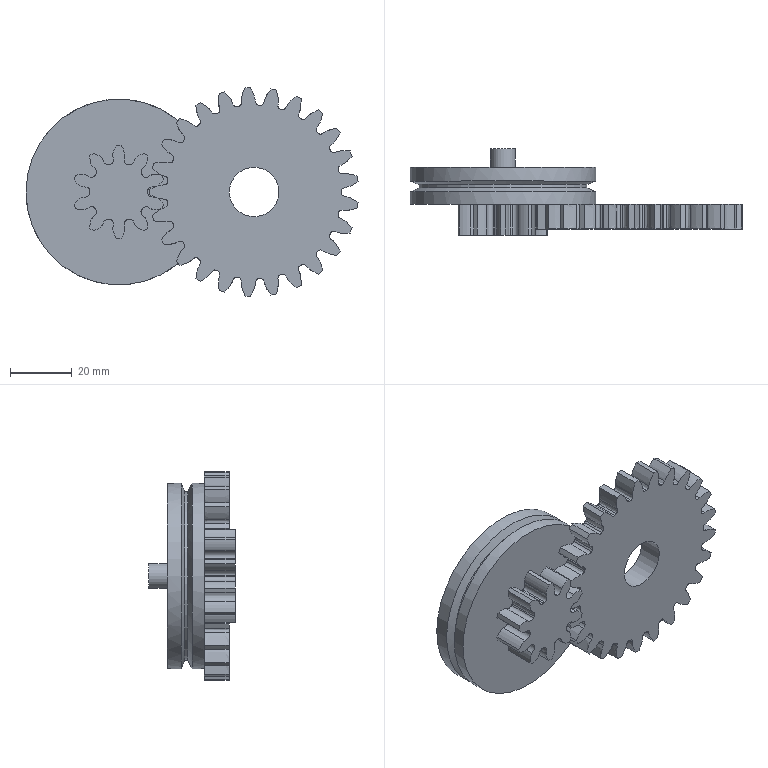Component | NX | MODEL6 | 3 solids | 224 faces | volume 60347 mm3 | other 125 | spline 50 | cylinder 40 | plane 7 | cone 2 | commonest cylinder face diameters 56.25 x25 18.71 x10 60 x2 8 x1 54.423 x1 16 x1